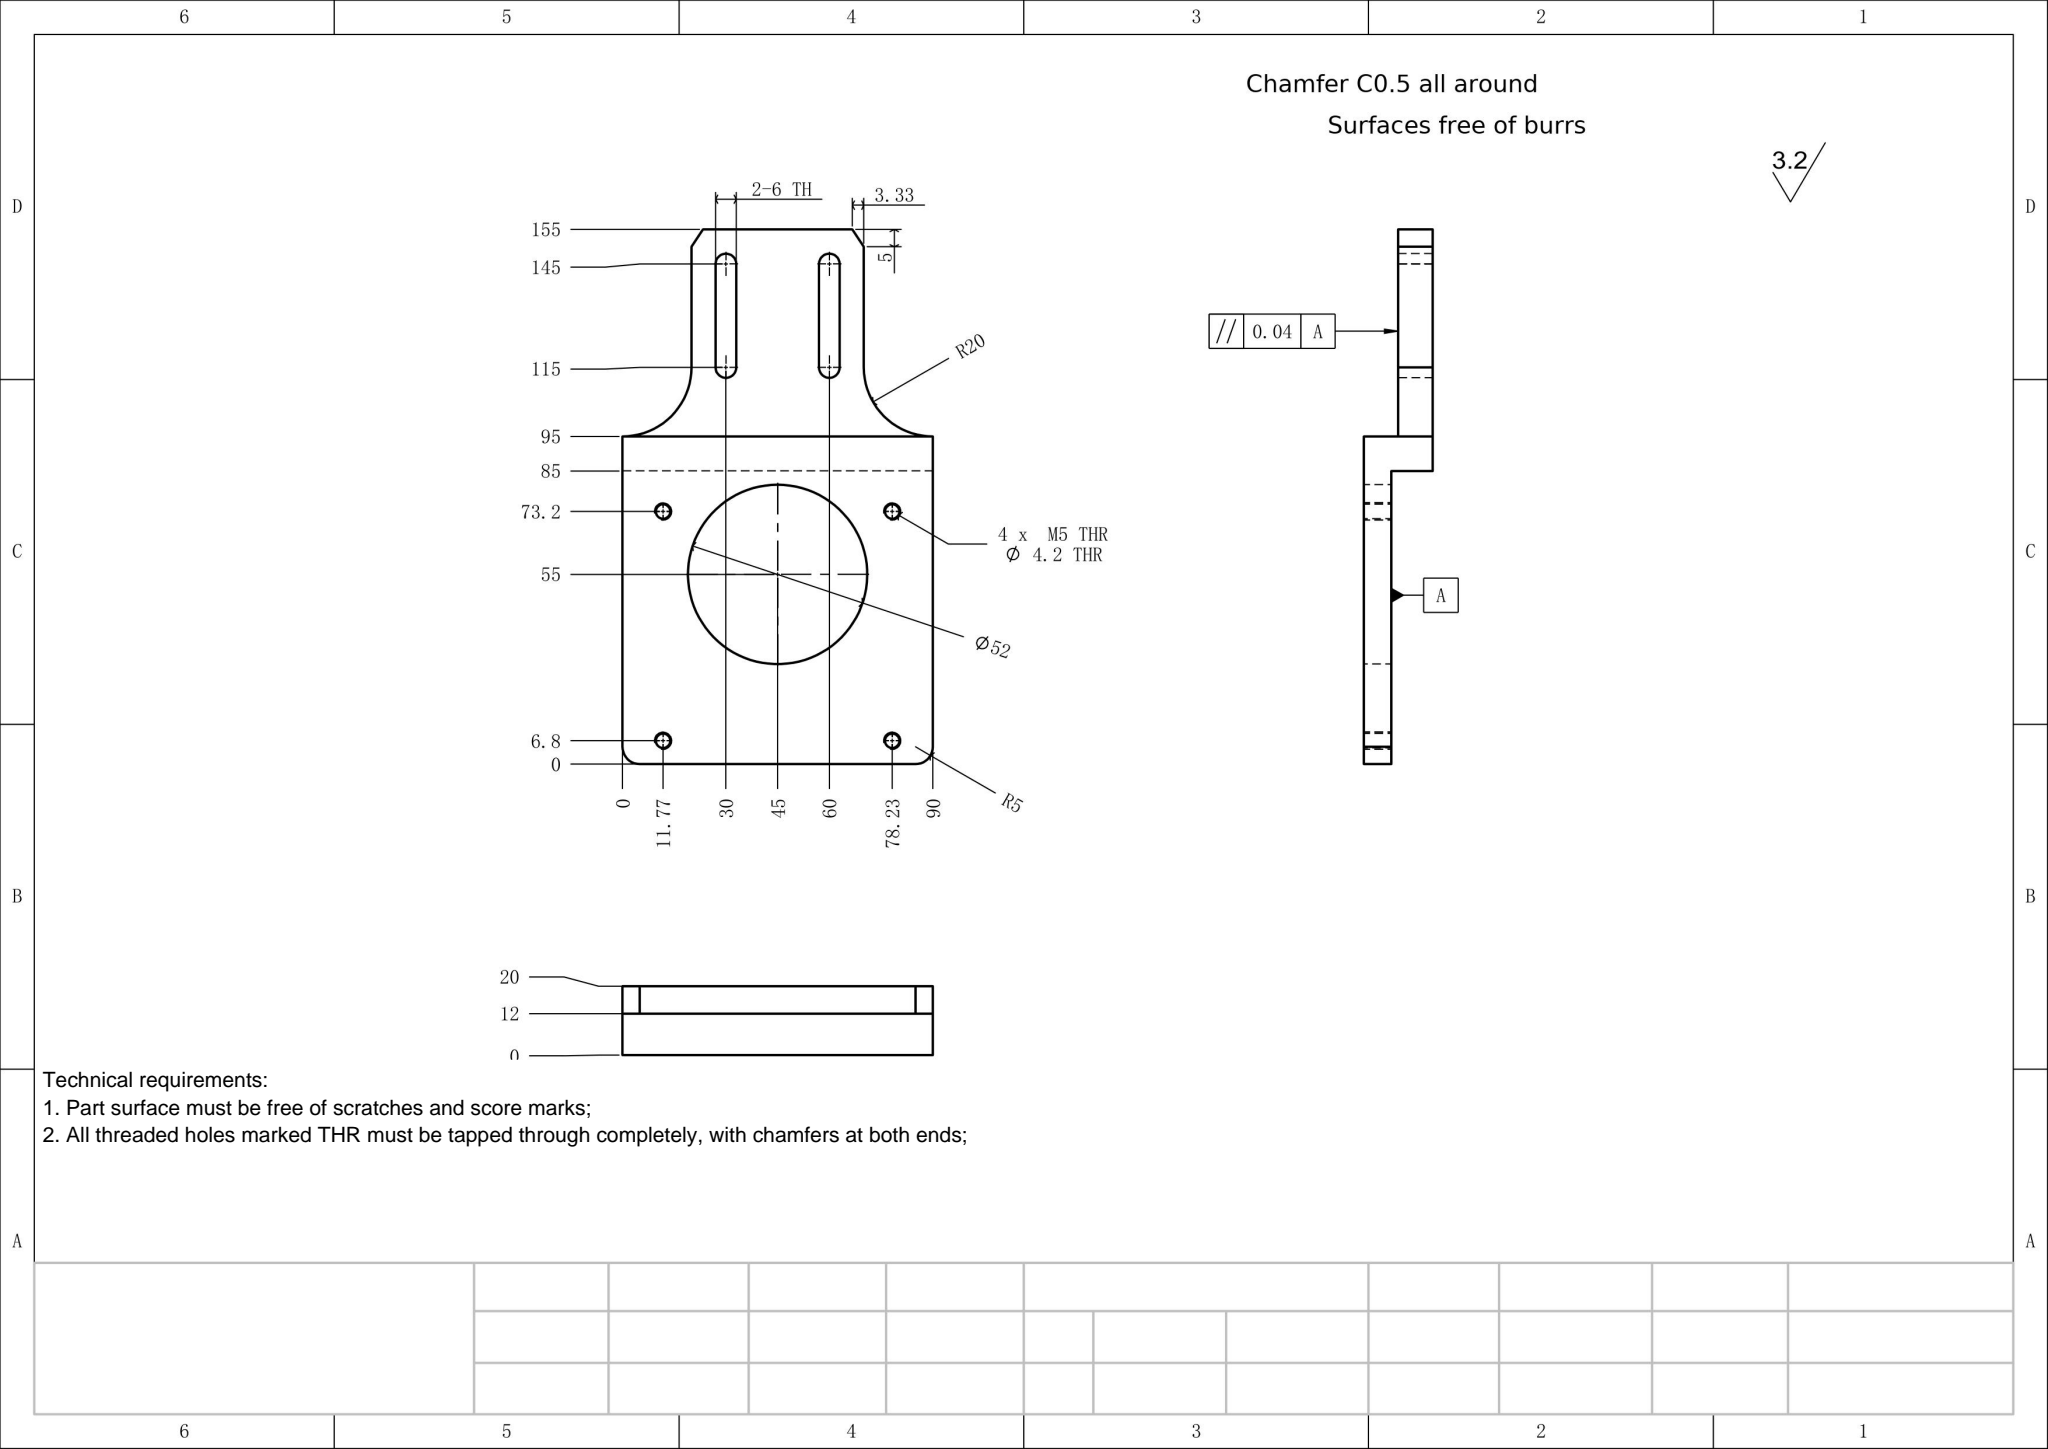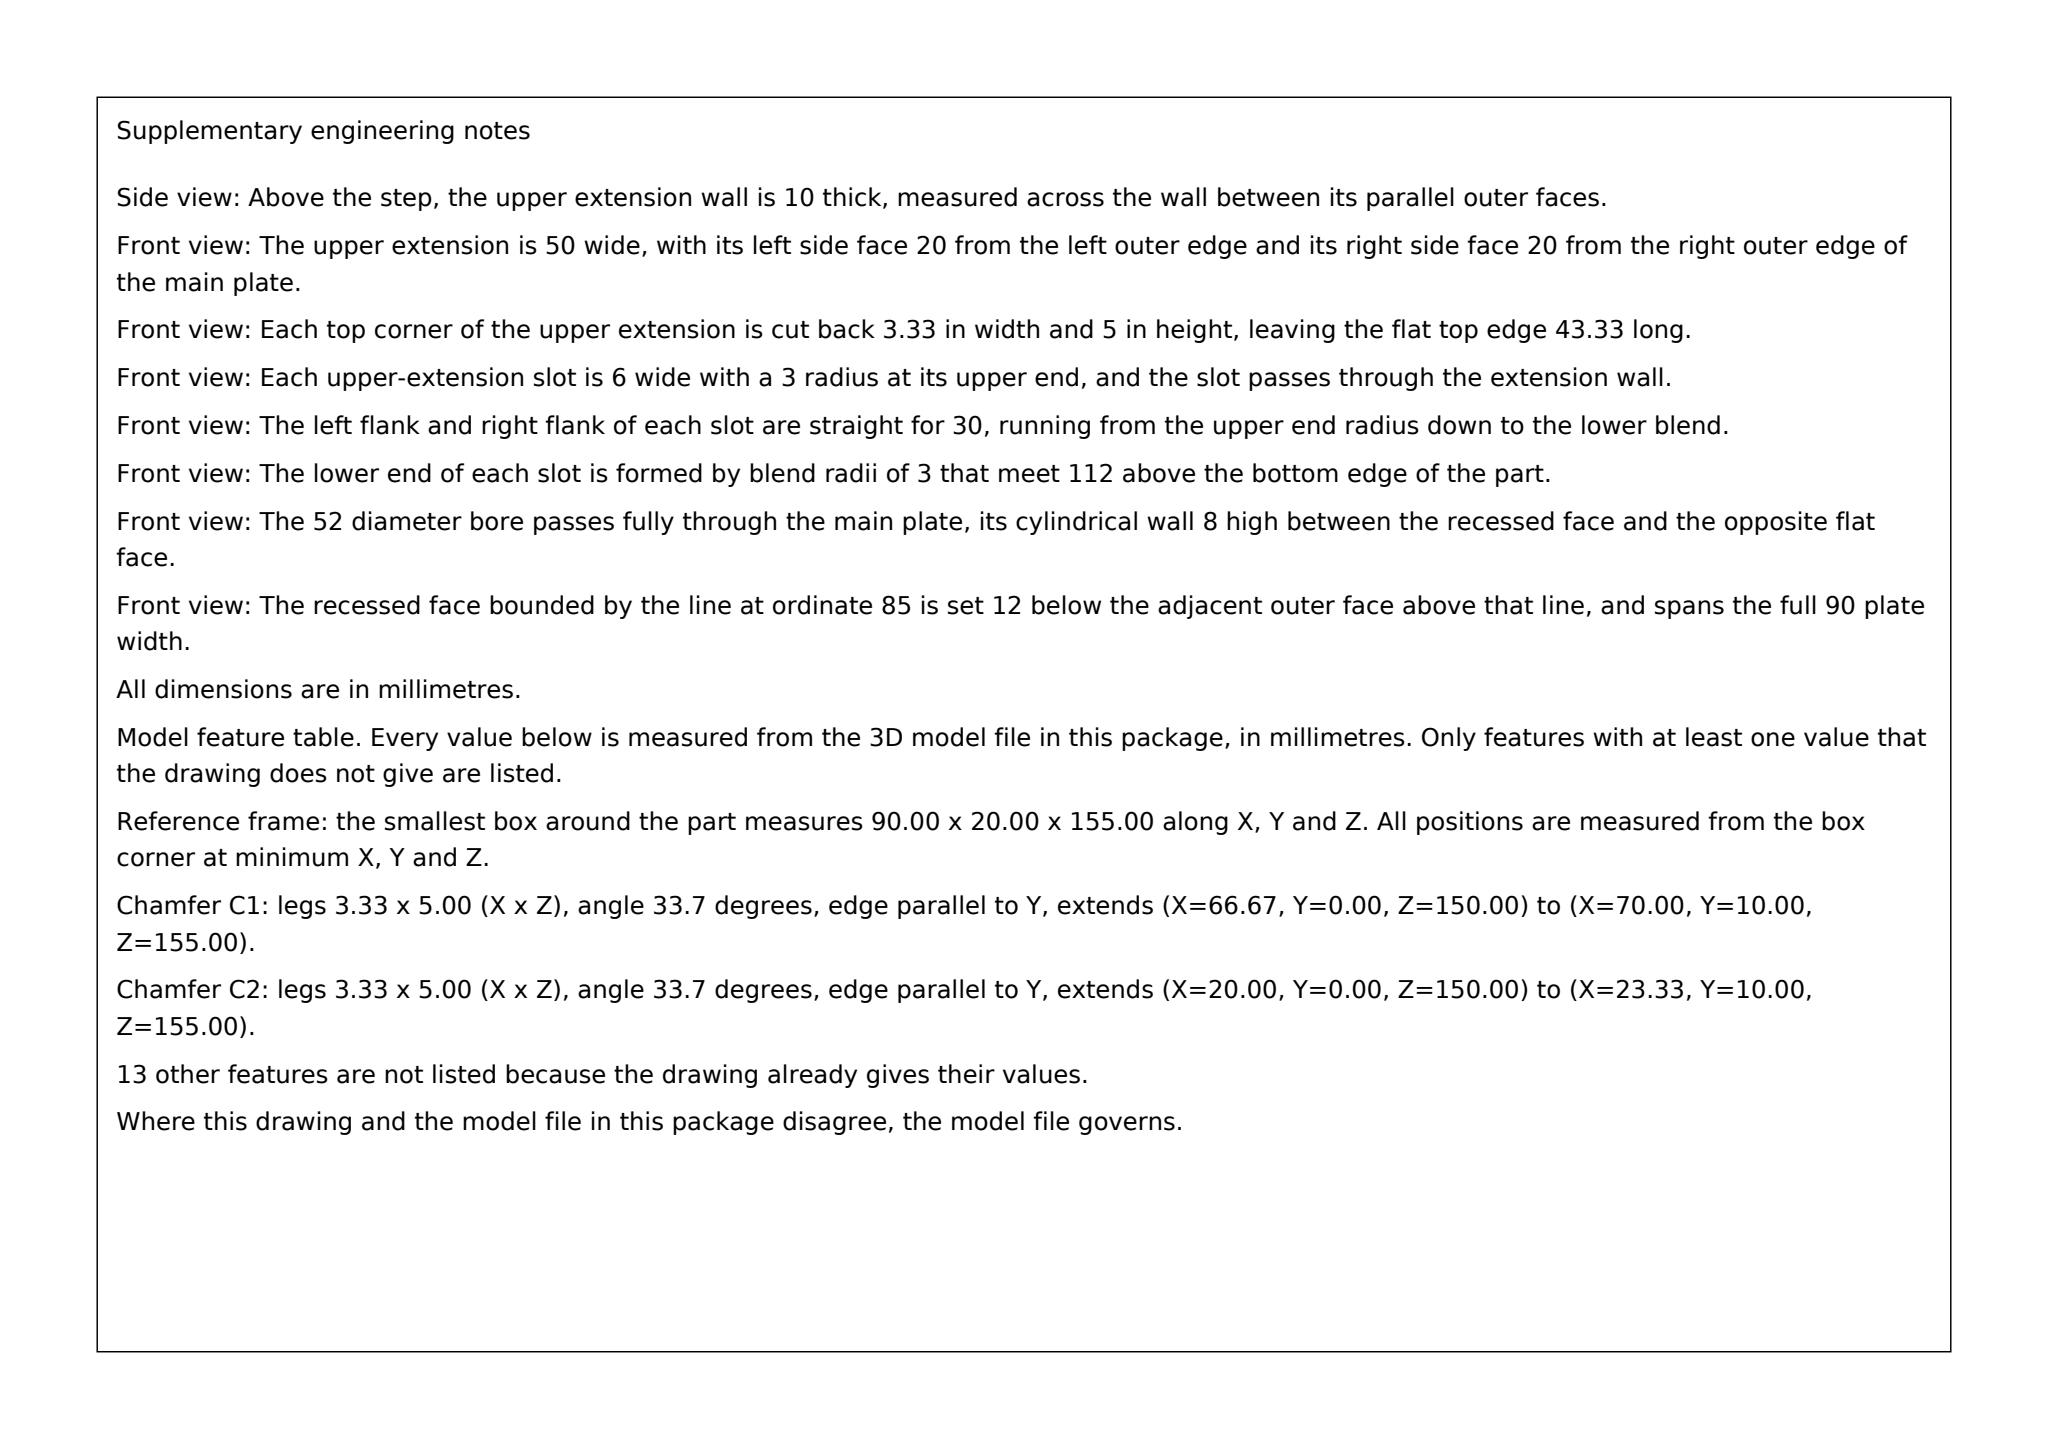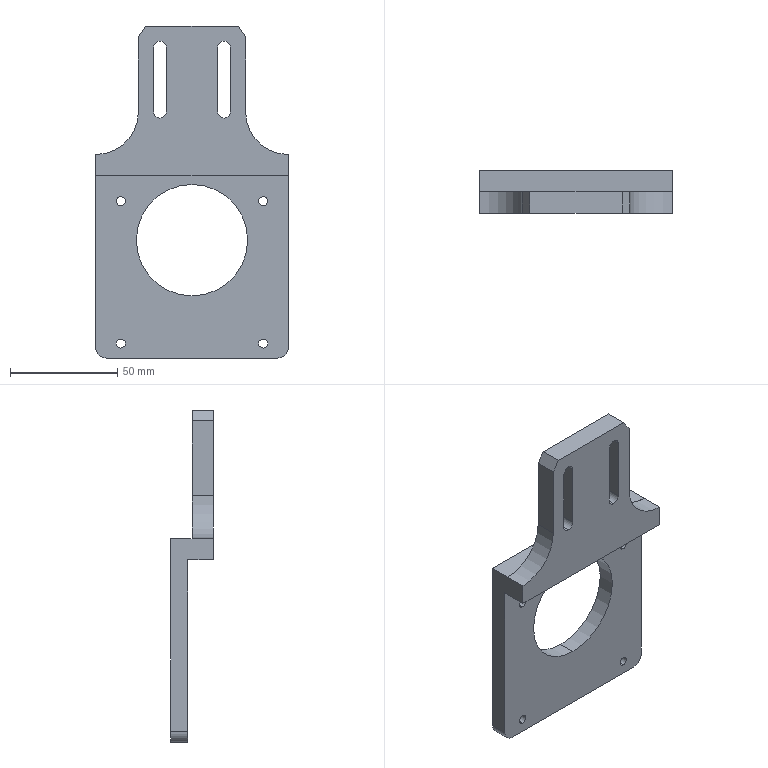Part | SolidWorks | mm | 1 solid | 38 faces | box 90 x 20 x 155 mm | volume 89066 mm3 | cylinder 20 | plane 18 | commonest cylinder face diameters 4.2 x8 6 x6 52 x2 10 x2 40 x2
Drawing notes:
Upper (neck) slab thickness: 10 mm, measured from the back face (datum A, y = 0) to y = 10; applies to the portion above z = 95. | from the solid: axis_planes[y,0.0] and axis_planes[y,10.0]; neck features (Ø6 slots, R20) are 10 mm deep in y
All dimensions in millimeters (mm) unless otherwise stated. | from the solid: STEP model facts units: mm
NECK (UPPER) SLAB THICKNESS 10 mm: REAR FACE Y=0 TO FRONT FACE Y=10, APPLIES OVER Z=95 TO 155 (TOP NECK REGION) | from the solid: axis_planes normal y at offset 0.0 and 10.0; bbox_xyz y=20 overall with step faces y=12/20 at lower slab
ALL DIMENSIONS IN MILLIMETERS | from the solid: STEP model facts stated in mm
NECK WIDTH 50 (X=20 TO X=70), SYMMETRIC ABOUT X=45, OVER Z=95 TO Z=155 | from the solid: axis_planes x=20 and x=70 (with z planes 95 and 155); neck blend cylinders dia 40 at x=0 and x=90, z=115
NECK (UPPER) SLAB THICKNESS 10: FROM DATUM A (Y=0) TO Y=10, OVER Z=95 TO Z=155 | from the solid: axis_planes y=0 and y=10; dia 40 and dia 6 cylinders at z=115/145 have length 10 along y
OVERALL BASE THICKNESS 20 FROM DATUM A (Y=0) TO Y=20, OVER Z=0 TO Z=95; STEP FACE AT Y=12 | from the solid: axis_planes y=0, y=12, y=20; bbox_xyz y=20; z planes 0 and 95
Ø52 BORE AXIS LOCATED AT X=45, Z=55 FROM BBOX MIN CORNER, AXIS PARALLEL TO Y (NORMAL TO DATUM A) | from the solid: cylinders[52, axis y, pos (45, 55)]
NECK (UPPER) SLAB THICKNESS 10 FROM DATUM A (Y=0) TO Y=10, OVER Z=95 TO Z=155 | from the solid: axis_planes y=0 (x 0-90, z 85-155) and y=10 (x 0-90, z 95-155)